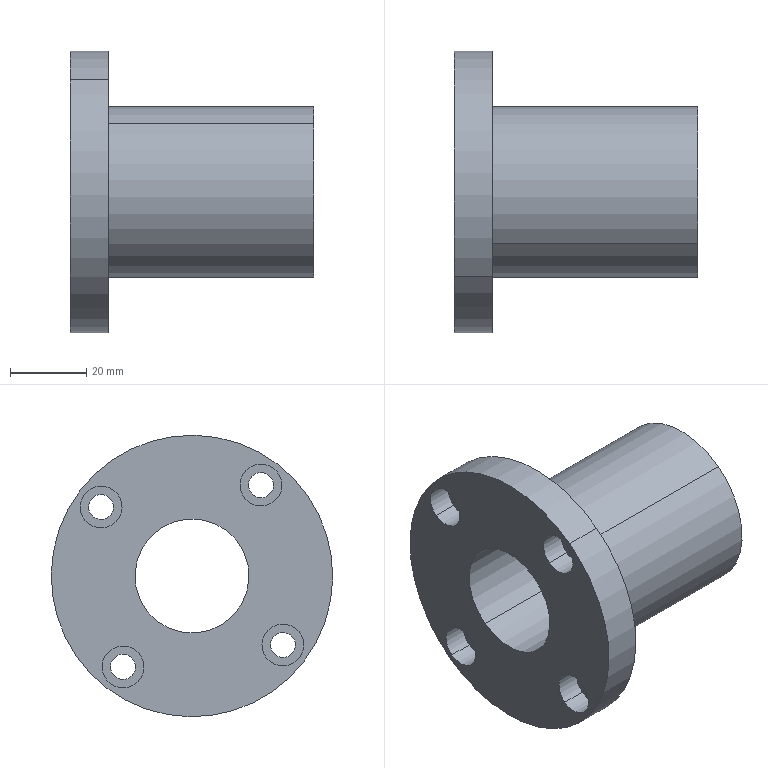Component | SolidWorks | 30LinearBearing-1 | 1 solid | 29 faces | box 64 x 74 x 74 mm | volume 80703 mm3 | cylinder 22 | plane 7 | commonest cylinder face diameters 11 x8 6.6 x8 45 x2 74 x2 30 x2
STEP:
#1=COLOUR_RGB('',0.7922,0.8196,0.9333);
#2=FILL_AREA_STYLE_COLOUR('',#1);
#3=FILL_AREA_STYLE('',(#2));
#4=SURFACE_STYLE_FILL_AREA(#3);
#5=SURFACE_SIDE_STYLE('',(#4));
#6=SURFACE_STYLE_USAGE(.BOTH.,#5);
#7=PRESENTATION_STYLE_ASSIGNMENT((#6));
#8=CARTESIAN_POINT('',(20.217,52.014,25.938));
#9=VERTEX_POINT('',#8);
#10=CARTESIAN_POINT('',(20.217,51.753,26.283));
#11=VERTEX_POINT('',#10);
#12=CARTESIAN_POINT('',(20.217,51.883,26.111));
#13=DIRECTION('',(-1.,-0.,-0.));
#14=DIRECTION('',(0.,-0.6045,0.7966));
#15=AXIS2_PLACEMENT_3D('',#12,#13,#14);
#16=CIRCLE('',#15,0.2165);
#17=EDGE_CURVE('',#9,#11,#16,.T.);
#18=ORIENTED_EDGE('',*,*,#17,.F.);
#19=CARTESIAN_POINT('',(19.961,52.014,25.938));
#20=VERTEX_POINT('',#19);
#21=CARTESIAN_POINT('',(20.217,52.014,25.938));
#22=DIRECTION('',(-1.,-0.,-0.));
#23=VECTOR('',#22,39.37);
#24=LINE('',#21,#23);
#25=EDGE_CURVE('',#9,#20,#24,.T.);
#26=ORIENTED_EDGE('',*,*,#25,.T.);
#27=CARTESIAN_POINT('',(19.961,51.753,26.283));
#28=VERTEX_POINT('',#27);
#29=CARTESIAN_POINT('',(19.961,51.883,26.111));
#30=DIRECTION('',(-1.,-0.,-0.));
#31=DIRECTION('',(0.,-0.6045,0.7966));
#32=AXIS2_PLACEMENT_3D('',#29,#30,#31);
#33=CIRCLE('',#32,0.2165);
#34=EDGE_CURVE('',#20,#28,#33,.T.);
#35=ORIENTED_EDGE('',*,*,#34,.T.);
#36=CARTESIAN_POINT('',(20.217,51.753,26.283));
#37=DIRECTION('',(-1.,-0.,-0.));
#38=VECTOR('',#37,39.37);
#39=LINE('',#36,#38);
#40=EDGE_CURVE('',#11,#28,#39,.T.);
#41=ORIENTED_EDGE('',*,*,#40,.F.);
#42=EDGE_LOOP('',(#18,#26,#35,#41));
#43=FACE_OUTER_BOUND('',#42,.T.);
#44=CARTESIAN_POINT('',(20.217,51.883,26.111));
#45=DIRECTION('',(-1.,-0.,-0.));
#46=DIRECTION('',(0.,-0.6045,0.7966));
#47=AXIS2_PLACEMENT_3D('',#44,#45,#46);
#48=CYLINDRICAL_SURFACE('',#47,0.2165);
#49=ADVANCED_FACE('',(#43),#48,.F.);
#50=CARTESIAN_POINT('',(20.217,50.36,26.165));
#51=VERTEX_POINT('',#50);
#52=CARTESIAN_POINT('',(20.217,50.098,26.51));
#53=VERTEX_POINT('',#52);
#54=CARTESIAN_POINT('',(20.217,50.229,26.338));
#55=DIRECTION('',(-1.,-0.,-0.));
#56=DIRECTION('',(0.,-0.6045,0.7966));
#57=AXIS2_PLACEMENT_3D('',#54,#55,#56);
#58=CIRCLE('',#57,0.2165);
#59=EDGE_CURVE('',#51,#53,#58,.T.);
#60=ORIENTED_EDGE('',*,*,#59,.F.);
#61=CARTESIAN_POINT('',(19.961,50.36,26.165));
#62=VERTEX_POINT('',#61);
#63=CARTESIAN_POINT('',(20.217,50.36,26.165));
#64=DIRECTION('',(-1.,-0.,-0.));
#65=VECTOR('',#64,39.37);
#66=LINE('',#63,#65);
#67=EDGE_CURVE('',#51,#62,#66,.T.);
#68=ORIENTED_EDGE('',*,*,#67,.T.);
#69=CARTESIAN_POINT('',(19.961,50.098,26.51));
#70=VERTEX_POINT('',#69);
#71=CARTESIAN_POINT('',(19.961,50.229,26.338));
#72=DIRECTION('',(-1.,-0.,-0.));
#73=DIRECTION('',(0.,-0.6045,0.7966));
#74=AXIS2_PLACEMENT_3D('',#71,#72,#73);
#75=CIRCLE('',#74,0.2165);
#76=EDGE_CURVE('',#62,#70,#75,.T.);
#77=ORIENTED_EDGE('',*,*,#76,.T.);
#78=CARTESIAN_POINT('',(20.217,50.098,26.51));
#79=DIRECTION('',(-1.,-0.,-0.));
#80=VECTOR('',#79,39.37);
#81=LINE('',#78,#80);
#82=EDGE_CURVE('',#53,#70,#81,.T.);
#83=ORIENTED_EDGE('',*,*,#82,.F.);
#84=EDGE_LOOP('',(#60,#68,#77,#83));
#85=FACE_OUTER_BOUND('',#84,.T.);
#86=CARTESIAN_POINT('',(20.217,50.229,26.338));
#87=DIRECTION('',(-1.,-0.,-0.));
#88=DIRECTION('',(0.,-0.6045,0.7966));
#89=AXIS2_PLACEMENT_3D('',#86,#87,#88);
#90=CYLINDRICAL_SURFACE('',#89,0.2165);
#91=ADVANCED_FACE('',(#85),#90,.F.);
#92=CARTESIAN_POINT('',(20.217,50.586,27.82));
#93=VERTEX_POINT('',#92);
#94=CARTESIAN_POINT('',(20.217,50.325,28.165));
#95=VERTEX_POINT('',#94);
#96=CARTESIAN_POINT('',(20.217,50.456,27.993));
#97=DIRECTION('',(-1.,-0.,-0.));
#98=DIRECTION('',(0.,-0.6045,0.7966));
#99=AXIS2_PLACEMENT_3D('',#96,#97,#98);
#100=CIRCLE('',#99,0.2165);
#101=EDGE_CURVE('',#93,#95,#100,.T.);
#102=ORIENTED_EDGE('',*,*,#101,.F.);
#103=CARTESIAN_POINT('',(19.961,50.586,27.82));
#104=VERTEX_POINT('',#103);
#105=CARTESIAN_POINT('',(20.217,50.586,27.82));
#106=DIRECTION('',(-1.,-0.,-0.));
#107=VECTOR('',#106,39.37);
#108=LINE('',#105,#107);
#109=EDGE_CURVE('',#93,#104,#108,.T.);
#110=ORIENTED_EDGE('',*,*,#109,.T.);
#111=CARTESIAN_POINT('',(19.961,50.325,28.165));
#112=VERTEX_POINT('',#111);
#113=CARTESIAN_POINT('',(19.961,50.456,27.993));
#114=DIRECTION('',(-1.,-0.,-0.));
#115=DIRECTION('',(0.,-0.6045,0.7966));
#116=AXIS2_PLACEMENT_3D('',#113,#114,#115);
#117=CIRCLE('',#116,0.2165);
#118=EDGE_CURVE('',#104,#112,#117,.T.);
#119=ORIENTED_EDGE('',*,*,#118,.T.);
#120=CARTESIAN_POINT('',(20.217,50.325,28.165));
#121=DIRECTION('',(-1.,-0.,-0.));
#122=VECTOR('',#121,39.37);
#123=LINE('',#120,#122);
#124=EDGE_CURVE('',#95,#112,#123,.T.);
#125=ORIENTED_EDGE('',*,*,#124,.F.);
#126=EDGE_LOOP('',(#102,#110,#119,#125));
#127=FACE_OUTER_BOUND('',#126,.T.);
#128=CARTESIAN_POINT('',(20.217,50.456,27.993));
#129=DIRECTION('',(-1.,-0.,-0.));
#130=DIRECTION('',(0.,-0.6045,0.7966));
#131=AXIS2_PLACEMENT_3D('',#128,#129,#130);
#132=CYLINDRICAL_SURFACE('',#131,0.2165);
#133=ADVANCED_FACE('',(#127),#132,.F.);
#134=CARTESIAN_POINT('',(20.217,52.241,27.593));
#135=VERTEX_POINT('',#134);
#136=CARTESIAN_POINT('',(20.217,51.98,27.938));
#137=VERTEX_POINT('',#136);
#138=CARTESIAN_POINT('',(20.217,52.11,27.766));
#139=DIRECTION('',(-1.,-0.,-0.));
#140=DIRECTION('',(0.,-0.6045,0.7966));
#141=AXIS2_PLACEMENT_3D('',#138,#139,#140);
#142=CIRCLE('',#141,0.2165);
#143=EDGE_CURVE('',#135,#137,#142,.T.);
#144=ORIENTED_EDGE('',*,*,#143,.F.);
#145=CARTESIAN_POINT('',(19.961,52.241,27.593));
#146=VERTEX_POINT('',#145);
#147=CARTESIAN_POINT('',(20.217,52.241,27.593));
#148=DIRECTION('',(-1.,-0.,-0.));
#149=VECTOR('',#148,39.37);
#150=LINE('',#147,#149);
#151=EDGE_CURVE('',#135,#146,#150,.T.);
#152=ORIENTED_EDGE('',*,*,#151,.T.);
#153=CARTESIAN_POINT('',(19.961,51.98,27.938));
#154=VERTEX_POINT('',#153);
#155=CARTESIAN_POINT('',(19.961,52.11,27.766));
#156=DIRECTION('',(-1.,-0.,-0.));
#157=DIRECTION('',(0.,-0.6045,0.7966));
#158=AXIS2_PLACEMENT_3D('',#155,#156,#157);
#159=CIRCLE('',#158,0.2165);
#160=EDGE_CURVE('',#146,#154,#159,.T.);
#161=ORIENTED_EDGE('',*,*,#160,.T.);
#162=CARTESIAN_POINT('',(20.217,51.98,27.938));
#163=DIRECTION('',(-1.,-0.,-0.));
#164=VECTOR('',#163,39.37);
#165=LINE('',#162,#164);
#166=EDGE_CURVE('',#137,#154,#165,.T.);
#167=ORIENTED_EDGE('',*,*,#166,.F.);
#168=EDGE_LOOP('',(#144,#152,#161,#167));
#169=FACE_OUTER_BOUND('',#168,.T.);
#170=CARTESIAN_POINT('',(20.217,52.11,27.766));
#171=DIRECTION('',(-1.,-0.,-0.));
#172=DIRECTION('',(0.,-0.6045,0.7966));
#173=AXIS2_PLACEMENT_3D('',#170,#171,#172);
#174=CYLINDRICAL_SURFACE('',#173,0.2165);
#175=ADVANCED_FACE('',(#169),#174,.F.);
#176=CARTESIAN_POINT('',(22.48,50.634,27.757));
#177=VERTEX_POINT('',#176);
#178=CARTESIAN_POINT('',(22.48,51.705,26.346));
#179=VERTEX_POINT('',#178);
#180=CARTESIAN_POINT('',(22.48,51.17,27.052));
#181=DIRECTION('',(-1.,-0.,-0.));
#182=DIRECTION('',(0.,-0.6045,0.7966));
#183=AXIS2_PLACEMENT_3D('',#180,#181,#182);
#184=CIRCLE('',#183,0.8858);
#185=EDGE_CURVE('',#177,#179,#184,.T.);
#186=ORIENTED_EDGE('',*,*,#185,.T.);
#187=CARTESIAN_POINT('',(20.354,51.705,26.346));
#188=VERTEX_POINT('',#187);
#189=CARTESIAN_POINT('',(17.576,51.705,26.346));
#190=DIRECTION('',(-1.,-0.,-0.));
#191=VECTOR('',#190,39.37);
#192=LINE('',#189,#191);
#193=EDGE_CURVE('',#179,#188,#192,.T.);
#194=ORIENTED_EDGE('',*,*,#193,.T.);
#195=CARTESIAN_POINT('',(20.354,50.634,27.757));
#196=VERTEX_POINT('',#195);
#197=CARTESIAN_POINT('',(20.354,51.17,27.052));
#198=DIRECTION('',(-1.,-0.,-0.));
#199=DIRECTION('',(0.,-0.6045,0.7966));
#200=AXIS2_PLACEMENT_3D('',#197,#198,#199);
#201=CIRCLE('',#200,0.8858);
#202=EDGE_CURVE('',#196,#188,#201,.T.);
#203=ORIENTED_EDGE('',*,*,#202,.F.);
#204=CARTESIAN_POINT('',(17.576,50.634,27.757));
#205=DIRECTION('',(-1.,-0.,-0.));
#206=VECTOR('',#205,39.37);
#207=LINE('',#204,#206);
#208=EDGE_CURVE('',#177,#196,#207,.T.);
#209=ORIENTED_EDGE('',*,*,#208,.F.);
#210=EDGE_LOOP('',(#186,#194,#203,#209));
#211=FACE_OUTER_BOUND('',#210,.T.);
#212=CARTESIAN_POINT('',(17.576,51.17,27.052));
#213=DIRECTION('',(-1.,-0.,-0.));
#214=DIRECTION('',(0.,-0.6045,0.7966));
#215=AXIS2_PLACEMENT_3D('',#212,#213,#214);
#216=CYLINDRICAL_SURFACE('',#215,0.8858);
#217=ADVANCED_FACE('',(#211),#216,.T.);
#218=CARTESIAN_POINT('',(20.354,50.289,28.212));
#219=VERTEX_POINT('',#218);
#220=CARTESIAN_POINT('',(20.354,52.05,25.891));
#221=VERTEX_POINT('',#220);
#222=CARTESIAN_POINT('',(20.354,51.17,27.052));
#223=DIRECTION('',(-1.,-0.,-0.));
#224=DIRECTION('',(0.,-0.6045,0.7966));
#225=AXIS2_PLACEMENT_3D('',#222,#223,#224);
#226=CIRCLE('',#225,1.457);
#227=EDGE_CURVE('',#219,#221,#226,.T.);
#228=ORIENTED_EDGE('',*,*,#227,.T.);
#229=CARTESIAN_POINT('',(19.961,52.05,25.891));
#230=VERTEX_POINT('',#229);
#231=CARTESIAN_POINT('',(17.576,52.05,25.891));
#232=DIRECTION('',(-1.,-0.,-0.));
#233=VECTOR('',#232,39.37);
#234=LINE('',#231,#233);
#235=EDGE_CURVE('',#221,#230,#234,.T.);
#236=ORIENTED_EDGE('',*,*,#235,.T.);
#237=CARTESIAN_POINT('',(19.961,50.289,28.212));
#238=VERTEX_POINT('',#237);
#239=CARTESIAN_POINT('',(19.961,51.17,27.052));
#240=DIRECTION('',(-1.,-0.,-0.));
#241=DIRECTION('',(0.,-0.6045,0.7966));
#242=AXIS2_PLACEMENT_3D('',#239,#240,#241);
#243=CIRCLE('',#242,1.457);
#244=EDGE_CURVE('',#238,#230,#243,.T.);
#245=ORIENTED_EDGE('',*,*,#244,.F.);
#246=CARTESIAN_POINT('',(17.576,50.289,28.212));
#247=DIRECTION('',(-1.,-0.,-0.));
#248=VECTOR('',#247,39.37);
#249=LINE('',#246,#248);
#250=EDGE_CURVE('',#219,#238,#249,.T.);
#251=ORIENTED_EDGE('',*,*,#250,.F.);
#252=EDGE_LOOP('',(#228,#236,#245,#251));
#253=FACE_OUTER_BOUND('',#252,.T.);
#254=CARTESIAN_POINT('',(17.576,51.17,27.052));
#255=DIRECTION('',(-1.,-0.,-0.));
#256=DIRECTION('',(0.,-0.6045,0.7966));
#257=AXIS2_PLACEMENT_3D('',#254,#255,#256);
#258=CYLINDRICAL_SURFACE('',#257,1.457);
#259=ADVANCED_FACE('',(#253),#258,.T.);
#260=CARTESIAN_POINT('',(22.48,51.526,26.581));
#261=VERTEX_POINT('',#260);
#262=CARTESIAN_POINT('',(22.48,50.813,27.522));
#263=VERTEX_POINT('',#262);
#264=CARTESIAN_POINT('',(22.48,51.17,27.052));
#265=DIRECTION('',(-1.,-0.,-0.));
#266=DIRECTION('',(0.,-0.6045,0.7966));
#267=AXIS2_PLACEMENT_3D('',#264,#265,#266);
#268=CIRCLE('',#267,0.5906);
#269=EDGE_CURVE('',#261,#263,#268,.T.);
#270=ORIENTED_EDGE('',*,*,#269,.F.);
#271=CARTESIAN_POINT('',(19.961,51.526,26.581));
#272=VERTEX_POINT('',#271);
#273=CARTESIAN_POINT('',(17.576,51.526,26.581));
#274=DIRECTION('',(-1.,-0.,-0.));
#275=VECTOR('',#274,39.37);
#276=LINE('',#273,#275);
#277=EDGE_CURVE('',#261,#272,#276,.T.);
#278=ORIENTED_EDGE('',*,*,#277,.T.);
#279=CARTESIAN_POINT('',(19.961,50.813,27.522));
#280=VERTEX_POINT('',#279);
#281=CARTESIAN_POINT('',(19.961,51.17,27.052));
#282=DIRECTION('',(-1.,-0.,-0.));
#283=DIRECTION('',(0.,-0.6045,0.7966));
#284=AXIS2_PLACEMENT_3D('',#281,#282,#283);
#285=CIRCLE('',#284,0.5906);
#286=EDGE_CURVE('',#272,#280,#285,.T.);
#287=ORIENTED_EDGE('',*,*,#286,.T.);
#288=CARTESIAN_POINT('',(17.576,50.813,27.522));
#289=DIRECTION('',(-1.,-0.,-0.));
#290=VECTOR('',#289,39.37);
#291=LINE('',#288,#290);
#292=EDGE_CURVE('',#263,#280,#291,.T.);
#293=ORIENTED_EDGE('',*,*,#292,.F.);
#294=EDGE_LOOP('',(#270,#278,#287,#293));
#295=FACE_OUTER_BOUND('',#294,.T.);
#296=CARTESIAN_POINT('',(17.576,51.17,27.052));
#297=DIRECTION('',(-1.,-0.,-0.));
#298=DIRECTION('',(0.,-0.6045,0.7966));
#299=AXIS2_PLACEMENT_3D('',#296,#297,#298);
#300=CYLINDRICAL_SURFACE('',#299,0.5906);
#301=ADVANCED_FACE('',(#295),#300,.F.);
#302=CARTESIAN_POINT('',(20.354,52.189,27.662));
#303=VERTEX_POINT('',#302);
#304=CARTESIAN_POINT('',(20.354,52.032,27.869));
#305=VERTEX_POINT('',#304);
#306=CARTESIAN_POINT('',(20.354,52.11,27.766));
#307=DIRECTION('',(-1.,-0.,-0.));
#308=DIRECTION('',(0.,-0.6045,0.7966));
#309=AXIS2_PLACEMENT_3D('',#306,#307,#308);
#310=CIRCLE('',#309,0.1299);
#311=EDGE_CURVE('',#303,#305,#310,.T.);
#312=ORIENTED_EDGE('',*,*,#311,.F.);
#313=CARTESIAN_POINT('',(20.217,52.189,27.662));
#314=VERTEX_POINT('',#313);
#315=CARTESIAN_POINT('',(22.48,52.189,27.662));
#316=DIRECTION('',(-1.,-0.,-0.));
#317=VECTOR('',#316,39.37);
#318=LINE('',#315,#317);
#319=EDGE_CURVE('',#303,#314,#318,.T.);
#320=ORIENTED_EDGE('',*,*,#319,.T.);
#321=CARTESIAN_POINT('',(20.217,52.032,27.869));
#322=VERTEX_POINT('',#321);
#323=CARTESIAN_POINT('',(20.217,52.11,27.766));
#324=DIRECTION('',(1.,0.,0.));
#325=DIRECTION('',(0.,-0.6045,0.7966));
#326=AXIS2_PLACEMENT_3D('',#323,#324,#325);
#327=CIRCLE('',#326,0.1299);
#328=EDGE_CURVE('',#322,#314,#327,.T.);
#329=ORIENTED_EDGE('',*,*,#328,.F.);
#330=CARTESIAN_POINT('',(22.48,52.032,27.869));
#331=DIRECTION('',(-1.,-0.,-0.));
#332=VECTOR('',#331,39.37);
#333=LINE('',#330,#332);
#334=EDGE_CURVE('',#305,#322,#333,.T.);
#335=ORIENTED_EDGE('',*,*,#334,.F.);
#336=EDGE_LOOP('',(#312,#320,#329,#335));
#337=FACE_OUTER_BOUND('',#336,.T.);
#338=CARTESIAN_POINT('',(22.48,52.11,27.766));
#339=DIRECTION('',(-1.,-0.,-0.));
#340=DIRECTION('',(0.,-0.6045,0.7966));
#341=AXIS2_PLACEMENT_3D('',#338,#339,#340);
#342=CYLINDRICAL_SURFACE('',#341,0.1299);
#343=ADVANCED_FACE('',(#337),#342,.F.);
#344=CARTESIAN_POINT('',(20.354,50.534,27.889));
#345=VERTEX_POINT('',#344);
#346=CARTESIAN_POINT('',(20.354,50.377,28.096));
#347=VERTEX_POINT('',#346);
#348=CARTESIAN_POINT('',(20.354,50.456,27.993));
#349=DIRECTION('',(-1.,-0.,-0.));
#350=DIRECTION('',(0.,-0.6045,0.7966));
#351=AXIS2_PLACEMENT_3D('',#348,#349,#350);
#352=CIRCLE('',#351,0.1299);
#353=EDGE_CURVE('',#345,#347,#352,.T.);
#354=ORIENTED_EDGE('',*,*,#353,.F.);
#355=CARTESIAN_POINT('',(20.217,50.534,27.889));
#356=VERTEX_POINT('',#355);
#357=CARTESIAN_POINT('',(22.48,50.534,27.889));
#358=DIRECTION('',(-1.,-0.,-0.));
#359=VECTOR('',#358,39.37);
#360=LINE('',#357,#359);
#361=EDGE_CURVE('',#345,#356,#360,.T.);
#362=ORIENTED_EDGE('',*,*,#361,.T.);
#363=CARTESIAN_POINT('',(20.217,50.377,28.096));
#364=VERTEX_POINT('',#363);
#365=CARTESIAN_POINT('',(20.217,50.456,27.993));
#366=DIRECTION('',(1.,0.,0.));
#367=DIRECTION('',(0.,-0.6045,0.7966));
#368=AXIS2_PLACEMENT_3D('',#365,#366,#367);
#369=CIRCLE('',#368,0.1299);
#370=EDGE_CURVE('',#364,#356,#369,.T.);
#371=ORIENTED_EDGE('',*,*,#370,.F.);
#372=CARTESIAN_POINT('',(22.48,50.377,28.096));
#373=DIRECTION('',(-1.,-0.,-0.));
#374=VECTOR('',#373,39.37);
#375=LINE('',#372,#374);
#376=EDGE_CURVE('',#347,#364,#375,.T.);
#377=ORIENTED_EDGE('',*,*,#376,.F.);
#378=EDGE_LOOP('',(#354,#362,#371,#377));
#379=FACE_OUTER_BOUND('',#378,.T.);
#380=CARTESIAN_POINT('',(22.48,50.456,27.993));
#381=DIRECTION('',(-1.,-0.,-0.));
#382=DIRECTION('',(0.,-0.6045,0.7966));
#383=AXIS2_PLACEMENT_3D('',#380,#381,#382);
#384=CYLINDRICAL_SURFACE('',#383,0.1299);
#385=ADVANCED_FACE('',(#379),#384,.F.);
#386=CARTESIAN_POINT('',(20.354,50.307,26.234));
#387=VERTEX_POINT('',#386);
#388=CARTESIAN_POINT('',(20.354,50.15,26.441));
#389=VERTEX_POINT('',#388);
#390=CARTESIAN_POINT('',(20.354,50.229,26.338));
#391=DIRECTION('',(-1.,-0.,-0.));
#392=DIRECTION('',(0.,-0.6045,0.7966));
#393=AXIS2_PLACEMENT_3D('',#390,#391,#392);
#394=CIRCLE('',#393,0.1299);
#395=EDGE_CURVE('',#387,#389,#394,.T.);
#396=ORIENTED_EDGE('',*,*,#395,.F.);
#397=CARTESIAN_POINT('',(20.217,50.307,26.234));
#398=VERTEX_POINT('',#397);
#399=CARTESIAN_POINT('',(22.48,50.307,26.234));
#400=DIRECTION('',(-1.,-0.,-0.));
#401=VECTOR('',#400,39.37);
#402=LINE('',#399,#401);
#403=EDGE_CURVE('',#387,#398,#402,.T.);
#404=ORIENTED_EDGE('',*,*,#403,.T.);
#405=CARTESIAN_POINT('',(20.217,50.15,26.441));
#406=VERTEX_POINT('',#405);
#407=CARTESIAN_POINT('',(20.217,50.229,26.338));
#408=DIRECTION('',(1.,0.,0.));
#409=DIRECTION('',(0.,-0.6045,0.7966));
#410=AXIS2_PLACEMENT_3D('',#407,#408,#409);
#411=CIRCLE('',#410,0.1299);
#412=EDGE_CURVE('',#406,#398,#411,.T.);
#413=ORIENTED_EDGE('',*,*,#412,.F.);
#414=CARTESIAN_POINT('',(22.48,50.15,26.441));
#415=DIRECTION('',(-1.,-0.,-0.));
#416=VECTOR('',#415,39.37);
#417=LINE('',#414,#416);
#418=EDGE_CURVE('',#389,#406,#417,.T.);
#419=ORIENTED_EDGE('',*,*,#418,.F.);
#420=EDGE_LOOP('',(#396,#404,#413,#419));
#421=FACE_OUTER_BOUND('',#420,.T.);
#422=CARTESIAN_POINT('',(22.48,50.229,26.338));
#423=DIRECTION('',(-1.,-0.,-0.));
#424=DIRECTION('',(0.,-0.6045,0.7966));
#425=AXIS2_PLACEMENT_3D('',#422,#423,#424);
#426=CYLINDRICAL_SURFACE('',#425,0.1299);
#427=ADVANCED_FACE('',(#421),#426,.F.);
#428=CARTESIAN_POINT('',(20.354,51.962,26.007));
#429=VERTEX_POINT('',#428);
#430=CARTESIAN_POINT('',(20.354,51.805,26.214));
#431=VERTEX_POINT('',#430);
#432=CARTESIAN_POINT('',(20.354,51.883,26.111));
#433=DIRECTION('',(-1.,-0.,-0.));
#434=DIRECTION('',(0.,-0.6045,0.7966));
#435=AXIS2_PLACEMENT_3D('',#432,#433,#434);
#436=CIRCLE('',#435,0.1299);
#437=EDGE_CURVE('',#429,#431,#436,.T.);
#438=ORIENTED_EDGE('',*,*,#437,.F.);
#439=CARTESIAN_POINT('',(20.217,51.962,26.007));
#440=VERTEX_POINT('',#439);
#441=CARTESIAN_POINT('',(22.48,51.962,26.007));
#442=DIRECTION('',(-1.,-0.,-0.));
#443=VECTOR('',#442,39.37);
#444=LINE('',#441,#443);
#445=EDGE_CURVE('',#429,#440,#444,.T.);
#446=ORIENTED_EDGE('',*,*,#445,.T.);
#447=CARTESIAN_POINT('',(20.217,51.805,26.214));
#448=VERTEX_POINT('',#447);
#449=CARTESIAN_POINT('',(20.217,51.883,26.111));
#450=DIRECTION('',(1.,0.,0.));
#451=DIRECTION('',(0.,-0.6045,0.7966));
#452=AXIS2_PLACEMENT_3D('',#449,#450,#451);
#453=CIRCLE('',#452,0.1299);
#454=EDGE_CURVE('',#448,#440,#453,.T.);
#455=ORIENTED_EDGE('',*,*,#454,.F.);
#456=CARTESIAN_POINT('',(22.48,51.805,26.214));
#457=DIRECTION('',(-1.,-0.,-0.));
#458=VECTOR('',#457,39.37);
#459=LINE('',#456,#458);
#460=EDGE_CURVE('',#431,#448,#459,.T.);
#461=ORIENTED_EDGE('',*,*,#460,.F.);
#462=EDGE_LOOP('',(#438,#446,#455,#461));
#463=FACE_OUTER_BOUND('',#462,.T.);
#464=CARTESIAN_POINT('',(22.48,51.883,26.111));
#465=DIRECTION('',(-1.,-0.,-0.));
#466=DIRECTION('',(0.,-0.6045,0.7966));
#467=AXIS2_PLACEMENT_3D('',#464,#465,#466);
#468=CYLINDRICAL_SURFACE('',#467,0.1299);
#469=ADVANCED_FACE('',(#463),#468,.F.);
#470=ORIENTED_EDGE('',*,*,#445,.F.);
#471=CARTESIAN_POINT('',(20.354,51.883,26.111));
#472=DIRECTION('',(-1.,-0.,-0.));
#473=DIRECTION('',(0.,-0.6045,0.7966));
#474=AXIS2_PLACEMENT_3D('',#471,#472,#473);
#475=CIRCLE('',#474,0.1299);
#476=EDGE_CURVE('',#431,#429,#475,.T.);
#477=ORIENTED_EDGE('',*,*,#476,.F.);
#478=ORIENTED_EDGE('',*,*,#460,.T.);
#479=CARTESIAN_POINT('',(20.217,51.883,26.111));
#480=DIRECTION('',(1.,0.,0.));
#481=DIRECTION('',(0.,-0.6045,0.7966));
#482=AXIS2_PLACEMENT_3D('',#479,#480,#481);
#483=CIRCLE('',#482,0.1299);
#484=EDGE_CURVE('',#440,#448,#483,.T.);
#485=ORIENTED_EDGE('',*,*,#484,.F.);
#486=EDGE_LOOP('',(#470,#477,#478,#485));
#487=FACE_OUTER_BOUND('',#486,.T.);
#488=CARTESIAN_POINT('',(22.48,51.883,26.111));
#489=DIRECTION('',(-1.,-0.,-0.));
#490=DIRECTION('',(0.,-0.6045,0.7966));
#491=AXIS2_PLACEMENT_3D('',#488,#489,#490);
#492=CYLINDRICAL_SURFACE('',#491,0.1299);
#493=ADVANCED_FACE('',(#487),#492,.F.);
#494=ORIENTED_EDGE('',*,*,#403,.F.);
#495=CARTESIAN_POINT('',(20.354,50.229,26.338));
#496=DIRECTION('',(-1.,-0.,-0.));
#497=DIRECTION('',(0.,-0.6045,0.7966));
#498=AXIS2_PLACEMENT_3D('',#495,#496,#497);
#499=CIRCLE('',#498,0.1299);
#500=EDGE_CURVE('',#389,#387,#499,.T.);
#501=ORIENTED_EDGE('',*,*,#500,.F.);
#502=ORIENTED_EDGE('',*,*,#418,.T.);
#503=CARTESIAN_POINT('',(20.217,50.229,26.338));
#504=DIRECTION('',(1.,0.,0.));
#505=DIRECTION('',(0.,-0.6045,0.7966));
#506=AXIS2_PLACEMENT_3D('',#503,#504,#505);
#507=CIRCLE('',#506,0.1299);
#508=EDGE_CURVE('',#398,#406,#507,.T.);
#509=ORIENTED_EDGE('',*,*,#508,.F.);
#510=EDGE_LOOP('',(#494,#501,#502,#509));
#511=FACE_OUTER_BOUND('',#510,.T.);
#512=CARTESIAN_POINT('',(22.48,50.229,26.338));
#513=DIRECTION('',(-1.,-0.,-0.));
#514=DIRECTION('',(0.,-0.6045,0.7966));
#515=AXIS2_PLACEMENT_3D('',#512,#513,#514);
#516=CYLINDRICAL_SURFACE('',#515,0.1299);
#517=ADVANCED_FACE('',(#511),#516,.F.);
#518=ORIENTED_EDGE('',*,*,#361,.F.);
#519=CARTESIAN_POINT('',(20.354,50.456,27.993));
#520=DIRECTION('',(-1.,-0.,-0.));
#521=DIRECTION('',(0.,-0.6045,0.7966));
#522=AXIS2_PLACEMENT_3D('',#519,#520,#521);
#523=CIRCLE('',#522,0.1299);
#524=EDGE_CURVE('',#347,#345,#523,.T.);
#525=ORIENTED_EDGE('',*,*,#524,.F.);
#526=ORIENTED_EDGE('',*,*,#376,.T.);
#527=CARTESIAN_POINT('',(20.217,50.456,27.993));
#528=DIRECTION('',(1.,0.,0.));
#529=DIRECTION('',(0.,-0.6045,0.7966));
#530=AXIS2_PLACEMENT_3D('',#527,#528,#529);
#531=CIRCLE('',#530,0.1299);
#532=EDGE_CURVE('',#356,#364,#531,.T.);
#533=ORIENTED_EDGE('',*,*,#532,.F.);
#534=EDGE_LOOP('',(#518,#525,#526,#533));
#535=FACE_OUTER_BOUND('',#534,.T.);
#536=CARTESIAN_POINT('',(22.48,50.456,27.993));
#537=DIRECTION('',(-1.,-0.,-0.));
#538=DIRECTION('',(0.,-0.6045,0.7966));
#539=AXIS2_PLACEMENT_3D('',#536,#537,#538);
#540=CYLINDRICAL_SURFACE('',#539,0.1299);
#541=ADVANCED_FACE('',(#535),#540,.F.);
#542=ORIENTED_EDGE('',*,*,#319,.F.);
#543=CARTESIAN_POINT('',(20.354,52.11,27.766));
#544=DIRECTION('',(-1.,-0.,-0.));
#545=DIRECTION('',(0.,-0.6045,0.7966));
#546=AXIS2_PLACEMENT_3D('',#543,#544,#545);
#547=CIRCLE('',#546,0.1299);
#548=EDGE_CURVE('',#305,#303,#547,.T.);
#549=ORIENTED_EDGE('',*,*,#548,.F.);
#550=ORIENTED_EDGE('',*,*,#334,.T.);
#551=CARTESIAN_POINT('',(20.217,52.11,27.766));
#552=DIRECTION('',(1.,0.,0.));
#553=DIRECTION('',(0.,-0.6045,0.7966));
#554=AXIS2_PLACEMENT_3D('',#551,#552,#553);
#555=CIRCLE('',#554,0.1299);
#556=EDGE_CURVE('',#314,#322,#555,.T.);
#557=ORIENTED_EDGE('',*,*,#556,.F.);
#558=EDGE_LOOP('',(#542,#549,#550,#557));
#559=FACE_OUTER_BOUND('',#558,.T.);
#560=CARTESIAN_POINT('',(22.48,52.11,27.766));
#561=DIRECTION('',(-1.,-0.,-0.));
#562=DIRECTION('',(0.,-0.6045,0.7966));
#563=AXIS2_PLACEMENT_3D('',#560,#561,#562);
#564=CYLINDRICAL_SURFACE('',#563,0.1299);
#565=ADVANCED_FACE('',(#559),#564,.F.);
#566=ORIENTED_EDGE('',*,*,#277,.F.);
#567=CARTESIAN_POINT('',(22.48,51.17,27.052));
#568=DIRECTION('',(-1.,-0.,-0.));
#569=DIRECTION('',(0.,-0.6045,0.7966));
#570=AXIS2_PLACEMENT_3D('',#567,#568,#569);
#571=CIRCLE('',#570,0.5906);
#572=EDGE_CURVE('',#263,#261,#571,.T.);
#573=ORIENTED_EDGE('',*,*,#572,.F.);
#574=ORIENTED_EDGE('',*,*,#292,.T.);
#575=CARTESIAN_POINT('',(19.961,51.17,27.052));
#576=DIRECTION('',(-1.,-0.,-0.));
#577=DIRECTION('',(0.,-0.6045,0.7966));
#578=AXIS2_PLACEMENT_3D('',#575,#576,#577);
#579=CIRCLE('',#578,0.5906);
#580=EDGE_CURVE('',#280,#272,#579,.T.);
#581=ORIENTED_EDGE('',*,*,#580,.T.);
#582=EDGE_LOOP('',(#566,#573,#574,#581));
#583=FACE_OUTER_BOUND('',#582,.T.);
#584=CARTESIAN_POINT('',(17.576,51.17,27.052));
#585=DIRECTION('',(-1.,-0.,-0.));
#586=DIRECTION('',(0.,-0.6045,0.7966));
#587=AXIS2_PLACEMENT_3D('',#584,#585,#586);
#588=CYLINDRICAL_SURFACE('',#587,0.5906);
#589=ADVANCED_FACE('',(#583),#588,.F.);
#590=CARTESIAN_POINT('',(19.961,51.883,26.111));
#591=DIRECTION('',(-1.,-0.,-0.));
#592=DIRECTION('',(0.,-0.6045,0.7966));
#593=AXIS2_PLACEMENT_3D('',#590,#591,#592);
#594=CIRCLE('',#593,0.2165);
#595=EDGE_CURVE('',#28,#20,#594,.T.);
#596=ORIENTED_EDGE('',*,*,#595,.F.);
#597=ORIENTED_EDGE('',*,*,#34,.F.);
#598=EDGE_LOOP('',(#596,#597));
#599=FACE_BOUND('',#598,.T.);
#600=CARTESIAN_POINT('',(19.961,50.229,26.338));
#601=DIRECTION('',(-1.,-0.,-0.));
#602=DIRECTION('',(0.,-0.6045,0.7966));
#603=AXIS2_PLACEMENT_3D('',#600,#601,#602);
#604=CIRCLE('',#603,0.2165);
#605=EDGE_CURVE('',#70,#62,#604,.T.);
#606=ORIENTED_EDGE('',*,*,#605,.F.);
#607=ORIENTED_EDGE('',*,*,#76,.F.);
#608=EDGE_LOOP('',(#606,#607));
#609=FACE_BOUND('',#608,.T.);
#610=CARTESIAN_POINT('',(19.961,50.456,27.993));
#611=DIRECTION('',(-1.,-0.,-0.));
#612=DIRECTION('',(0.,-0.6045,0.7966));
#613=AXIS2_PLACEMENT_3D('',#610,#611,#612);
#614=CIRCLE('',#613,0.2165);
#615=EDGE_CURVE('',#112,#104,#614,.T.);
#616=ORIENTED_EDGE('',*,*,#615,.F.);
#617=ORIENTED_EDGE('',*,*,#118,.F.);
#618=EDGE_LOOP('',(#616,#617));
#619=FACE_BOUND('',#618,.T.);
#620=CARTESIAN_POINT('',(19.961,52.11,27.766));
#621=DIRECTION('',(-1.,-0.,-0.));
#622=DIRECTION('',(0.,-0.6045,0.7966));
#623=AXIS2_PLACEMENT_3D('',#620,#621,#622);
#624=CIRCLE('',#623,0.2165);
#625=EDGE_CURVE('',#154,#146,#624,.T.);
#626=ORIENTED_EDGE('',*,*,#625,.F.);
#627=ORIENTED_EDGE('',*,*,#160,.F.);
#628=EDGE_LOOP('',(#626,#627));
#629=FACE_BOUND('',#628,.T.);
#630=ORIENTED_EDGE('',*,*,#580,.F.);
#631=ORIENTED_EDGE('',*,*,#286,.F.);
#632=EDGE_LOOP('',(#630,#631));
#633=FACE_BOUND('',#632,.T.);
#634=ORIENTED_EDGE('',*,*,#244,.T.);
#635=CARTESIAN_POINT('',(19.961,51.17,27.052));
#636=DIRECTION('',(-1.,-0.,-0.));
#637=DIRECTION('',(0.,-0.6045,0.7966));
#638=AXIS2_PLACEMENT_3D('',#635,#636,#637);
#639=CIRCLE('',#638,1.457);
#640=EDGE_CURVE('',#230,#238,#639,.T.);
#641=ORIENTED_EDGE('',*,*,#640,.T.);
#642=EDGE_LOOP('',(#634,#641));
#643=FACE_OUTER_BOUND('',#642,.T.);
#644=CARTESIAN_POINT('',(19.961,51.64,27.409));
#645=DIRECTION('',(1.,0.,0.));
#646=DIRECTION('',(-0.,0.6045,-0.7966));
#647=AXIS2_PLACEMENT_3D('',#644,#645,#646);
#648=PLANE('',#647);
#649=ADVANCED_FACE('',(#599,#609,#619,#629,#633,#643),#648,.F.);
#650=ORIENTED_EDGE('',*,*,#235,.F.);
#651=CARTESIAN_POINT('',(20.354,51.17,27.052));
#652=DIRECTION('',(-1.,-0.,-0.));
#653=DIRECTION('',(0.,-0.6045,0.7966));
#654=AXIS2_PLACEMENT_3D('',#651,#652,#653);
#655=CIRCLE('',#654,1.457);
#656=EDGE_CURVE('',#221,#219,#655,.T.);
#657=ORIENTED_EDGE('',*,*,#656,.T.);
#658=ORIENTED_EDGE('',*,*,#250,.T.);
#659=ORIENTED_EDGE('',*,*,#640,.F.);
#660=EDGE_LOOP('',(#650,#657,#658,#659));
#661=FACE_OUTER_BOUND('',#660,.T.);
#662=CARTESIAN_POINT('',(17.576,51.17,27.052));
#663=DIRECTION('',(-1.,-0.,-0.));
#664=DIRECTION('',(0.,-0.6045,0.7966));
#665=AXIS2_PLACEMENT_3D('',#662,#663,#664);
#666=CYLINDRICAL_SURFACE('',#665,1.457);
#667=ADVANCED_FACE('',(#661),#666,.T.);
#668=ORIENTED_EDGE('',*,*,#476,.T.);
#669=ORIENTED_EDGE('',*,*,#437,.T.);
#670=EDGE_LOOP('',(#668,#669));
#671=FACE_BOUND('',#670,.T.);
#672=ORIENTED_EDGE('',*,*,#500,.T.);
#673=ORIENTED_EDGE('',*,*,#395,.T.);
#674=EDGE_LOOP('',(#672,#673));
#675=FACE_BOUND('',#674,.T.);
#676=ORIENTED_EDGE('',*,*,#524,.T.);
#677=ORIENTED_EDGE('',*,*,#353,.T.);
#678=EDGE_LOOP('',(#676,#677));
#679=FACE_BOUND('',#678,.T.);
#680=ORIENTED_EDGE('',*,*,#548,.T.);
#681=ORIENTED_EDGE('',*,*,#311,.T.);
#682=EDGE_LOOP('',(#680,#681));
#683=FACE_BOUND('',#682,.T.);
#684=ORIENTED_EDGE('',*,*,#227,.F.);
#685=ORIENTED_EDGE('',*,*,#656,.F.);
#686=EDGE_LOOP('',(#684,#685));
#687=FACE_OUTER_BOUND('',#686,.T.);
#688=ORIENTED_EDGE('',*,*,#202,.T.);
#689=CARTESIAN_POINT('',(20.354,51.17,27.052));
#690=DIRECTION('',(-1.,-0.,-0.));
#691=DIRECTION('',(0.,-0.6045,0.7966));
#692=AXIS2_PLACEMENT_3D('',#689,#690,#691);
#693=CIRCLE('',#692,0.8858);
#694=EDGE_CURVE('',#188,#196,#693,.T.);
#695=ORIENTED_EDGE('',*,*,#694,.T.);
#696=EDGE_LOOP('',(#688,#695));
#697=FACE_BOUND('',#696,.T.);
#698=CARTESIAN_POINT('',(20.354,52.33,27.932));
#699=DIRECTION('',(-1.,-0.,-0.));
#700=DIRECTION('',(0.,-0.6045,0.7966));
#701=AXIS2_PLACEMENT_3D('',#698,#699,#700);
#702=PLANE('',#701);
#703=ADVANCED_FACE('',(#671,#675,#679,#683,#687,#697),#702,.F.);
#704=ORIENTED_EDGE('',*,*,#193,.F.);
#705=CARTESIAN_POINT('',(22.48,51.17,27.052));
#706=DIRECTION('',(-1.,-0.,-0.));
#707=DIRECTION('',(0.,-0.6045,0.7966));
#708=AXIS2_PLACEMENT_3D('',#705,#706,#707);
#709=CIRCLE('',#708,0.8858);
#710=EDGE_CURVE('',#179,#177,#709,.T.);
#711=ORIENTED_EDGE('',*,*,#710,.T.);
#712=ORIENTED_EDGE('',*,*,#208,.T.);
#713=ORIENTED_EDGE('',*,*,#694,.F.);
#714=EDGE_LOOP('',(#704,#711,#712,#713));
#715=FACE_OUTER_BOUND('',#714,.T.);
#716=CARTESIAN_POINT('',(17.576,51.17,27.052));
#717=DIRECTION('',(-1.,-0.,-0.));
#718=DIRECTION('',(0.,-0.6045,0.7966));
#719=AXIS2_PLACEMENT_3D('',#716,#717,#718);
#720=CYLINDRICAL_SURFACE('',#719,0.8858);
#721=ADVANCED_FACE('',(#715),#720,.T.);
#722=ORIENTED_EDGE('',*,*,#185,.F.);
#723=ORIENTED_EDGE('',*,*,#710,.F.);
#724=EDGE_LOOP('',(#722,#723));
#725=FACE_OUTER_BOUND('',#724,.T.);
#726=ORIENTED_EDGE('',*,*,#572,.T.);
#727=ORIENTED_EDGE('',*,*,#269,.T.);
#728=EDGE_LOOP('',(#726,#727));
#729=FACE_BOUND('',#728,.T.);
#730=CARTESIAN_POINT('',(22.48,51.875,27.587));
#731=DIRECTION('',(-1.,-0.,-0.));
#732=DIRECTION('',(0.,-0.6045,0.7966));
#733=AXIS2_PLACEMENT_3D('',#730,#731,#732);
#734=PLANE('',#733);
#735=ADVANCED_FACE('',(#725,#729),#734,.F.);
#736=CARTESIAN_POINT('',(20.217,52.11,27.766));
#737=DIRECTION('',(-1.,-0.,-0.));
#738=DIRECTION('',(0.,-0.6045,0.7966));
#739=AXIS2_PLACEMENT_3D('',#736,#737,#738);
#740=CIRCLE('',#739,0.2165);
#741=EDGE_CURVE('',#137,#135,#740,.T.);
#742=ORIENTED_EDGE('',*,*,#741,.T.);
#743=ORIENTED_EDGE('',*,*,#143,.T.);
#744=EDGE_LOOP('',(#742,#743));
#745=FACE_OUTER_BOUND('',#744,.T.);
#746=ORIENTED_EDGE('',*,*,#328,.T.);
#747=ORIENTED_EDGE('',*,*,#556,.T.);
#748=EDGE_LOOP('',(#746,#747));
#749=FACE_BOUND('',#748,.T.);
#750=CARTESIAN_POINT('',(20.217,52.11,27.766));
#751=DIRECTION('',(-1.,-0.,-0.));
#752=DIRECTION('',(0.,-0.6045,0.7966));
#753=AXIS2_PLACEMENT_3D('',#750,#751,#752);
#754=PLANE('',#753);
#755=ADVANCED_FACE('',(#745,#749),#754,.T.);
#756=ORIENTED_EDGE('',*,*,#151,.F.);
#757=ORIENTED_EDGE('',*,*,#741,.F.);
#758=ORIENTED_EDGE('',*,*,#166,.T.);
#759=ORIENTED_EDGE('',*,*,#625,.T.);
#760=EDGE_LOOP('',(#756,#757,#758,#759));
#761=FACE_OUTER_BOUND('',#760,.T.);
#762=CARTESIAN_POINT('',(20.217,52.11,27.766));
#763=DIRECTION('',(-1.,-0.,-0.));
#764=DIRECTION('',(0.,-0.6045,0.7966));
#765=AXIS2_PLACEMENT_3D('',#762,#763,#764);
#766=CYLINDRICAL_SURFACE('',#765,0.2165);
#767=ADVANCED_FACE('',(#761),#766,.F.);
#768=CARTESIAN_POINT('',(20.217,50.456,27.993));
#769=DIRECTION('',(-1.,-0.,-0.));
#770=DIRECTION('',(0.,-0.6045,0.7966));
#771=AXIS2_PLACEMENT_3D('',#768,#769,#770);
#772=CIRCLE('',#771,0.2165);
#773=EDGE_CURVE('',#95,#93,#772,.T.);
#774=ORIENTED_EDGE('',*,*,#773,.T.);
#775=ORIENTED_EDGE('',*,*,#101,.T.);
#776=EDGE_LOOP('',(#774,#775));
#777=FACE_OUTER_BOUND('',#776,.T.);
#778=ORIENTED_EDGE('',*,*,#370,.T.);
#779=ORIENTED_EDGE('',*,*,#532,.T.);
#780=EDGE_LOOP('',(#778,#779));
#781=FACE_BOUND('',#780,.T.);
#782=CARTESIAN_POINT('',(20.217,50.456,27.993));
#783=DIRECTION('',(-1.,-0.,-0.));
#784=DIRECTION('',(0.,-0.6045,0.7966));
#785=AXIS2_PLACEMENT_3D('',#782,#783,#784);
#786=PLANE('',#785);
#787=ADVANCED_FACE('',(#777,#781),#786,.T.);
#788=ORIENTED_EDGE('',*,*,#109,.F.);
#789=ORIENTED_EDGE('',*,*,#773,.F.);
#790=ORIENTED_EDGE('',*,*,#124,.T.);
#791=ORIENTED_EDGE('',*,*,#615,.T.);
#792=EDGE_LOOP('',(#788,#789,#790,#791));
#793=FACE_OUTER_BOUND('',#792,.T.);
#794=CARTESIAN_POINT('',(20.217,50.456,27.993));
#795=DIRECTION('',(-1.,-0.,-0.));
#796=DIRECTION('',(0.,-0.6045,0.7966));
#797=AXIS2_PLACEMENT_3D('',#794,#795,#796);
#798=CYLINDRICAL_SURFACE('',#797,0.2165);
#799=ADVANCED_FACE('',(#793),#798,.F.);
#800=CARTESIAN_POINT('',(20.217,50.229,26.338));
#801=DIRECTION('',(-1.,-0.,-0.));
#802=DIRECTION('',(0.,-0.6045,0.7966));
#803=AXIS2_PLACEMENT_3D('',#800,#801,#802);
#804=CIRCLE('',#803,0.2165);
#805=EDGE_CURVE('',#53,#51,#804,.T.);
#806=ORIENTED_EDGE('',*,*,#805,.T.);
#807=ORIENTED_EDGE('',*,*,#59,.T.);
#808=EDGE_LOOP('',(#806,#807));
#809=FACE_OUTER_BOUND('',#808,.T.);
#810=ORIENTED_EDGE('',*,*,#412,.T.);
#811=ORIENTED_EDGE('',*,*,#508,.T.);
#812=EDGE_LOOP('',(#810,#811));
#813=FACE_BOUND('',#812,.T.);
#814=CARTESIAN_POINT('',(20.217,50.229,26.338));
#815=DIRECTION('',(-1.,-0.,-0.));
#816=DIRECTION('',(0.,-0.6045,0.7966));
#817=AXIS2_PLACEMENT_3D('',#814,#815,#816);
#818=PLANE('',#817);
#819=ADVANCED_FACE('',(#809,#813),#818,.T.);
#820=ORIENTED_EDGE('',*,*,#67,.F.);
#821=ORIENTED_EDGE('',*,*,#805,.F.);
#822=ORIENTED_EDGE('',*,*,#82,.T.);
#823=ORIENTED_EDGE('',*,*,#605,.T.);
#824=EDGE_LOOP('',(#820,#821,#822,#823));
#825=FACE_OUTER_BOUND('',#824,.T.);
#826=CARTESIAN_POINT('',(20.217,50.229,26.338));
#827=DIRECTION('',(-1.,-0.,-0.));
#828=DIRECTION('',(0.,-0.6045,0.7966));
#829=AXIS2_PLACEMENT_3D('',#826,#827,#828);
#830=CYLINDRICAL_SURFACE('',#829,0.2165);
#831=ADVANCED_FACE('',(#825),#830,.F.);
#832=CARTESIAN_POINT('',(20.217,51.883,26.111));
#833=DIRECTION('',(-1.,-0.,-0.));
#834=DIRECTION('',(0.,-0.6045,0.7966));
#835=AXIS2_PLACEMENT_3D('',#832,#833,#834);
#836=CIRCLE('',#835,0.2165);
#837=EDGE_CURVE('',#11,#9,#836,.T.);
#838=ORIENTED_EDGE('',*,*,#837,.T.);
#839=ORIENTED_EDGE('',*,*,#17,.T.);
#840=EDGE_LOOP('',(#838,#839));
#841=FACE_OUTER_BOUND('',#840,.T.);
#842=ORIENTED_EDGE('',*,*,#454,.T.);
#843=ORIENTED_EDGE('',*,*,#484,.T.);
#844=EDGE_LOOP('',(#842,#843));
#845=FACE_BOUND('',#844,.T.);
#846=CARTESIAN_POINT('',(20.217,51.883,26.111));
#847=DIRECTION('',(-1.,-0.,-0.));
#848=DIRECTION('',(0.,-0.6045,0.7966));
#849=AXIS2_PLACEMENT_3D('',#846,#847,#848);
#850=PLANE('',#849);
#851=ADVANCED_FACE('',(#841,#845),#850,.T.);
#852=ORIENTED_EDGE('',*,*,#25,.F.);
#853=ORIENTED_EDGE('',*,*,#837,.F.);
#854=ORIENTED_EDGE('',*,*,#40,.T.);
#855=ORIENTED_EDGE('',*,*,#595,.T.);
#856=EDGE_LOOP('',(#852,#853,#854,#855));
#857=FACE_OUTER_BOUND('',#856,.T.);
#858=CARTESIAN_POINT('',(20.217,51.883,26.111));
#859=DIRECTION('',(-1.,-0.,-0.));
#860=DIRECTION('',(0.,-0.6045,0.7966));
#861=AXIS2_PLACEMENT_3D('',#858,#859,#860);
#862=CYLINDRICAL_SURFACE('',#861,0.2165);
#863=ADVANCED_FACE('',(#857),#862,.F.);
#864=CLOSED_SHELL('',(#49,#91,#133,#175,#217,#259,#301,#343,#385,#427,#469,#493,#517,#541,#565,#589,#649,#667,#703,#721,#735,#755,#767,#787,#799,#819,#831,#851,#863));
#865=MANIFOLD_SOLID_BREP('',#864);
#866=STYLED_ITEM('',(#7),#865);
#867=(LENGTH_UNIT()NAMED_UNIT(*)SI_UNIT($,.METRE.));
#868=LENGTH_MEASURE_WITH_UNIT(LENGTH_MEASURE(0.0254),#867);
#869=DIMENSIONAL_EXPONENTS(1.,0.,0.,0.,0.,0.,0.);
#870=(CONVERSION_BASED_UNIT('',#868)LENGTH_UNIT()NAMED_UNIT(#869));
#871=UNCERTAINTY_MEASURE_WITH_UNIT(LENGTH_MEASURE(0.00001),#870,'','');
#872=(NAMED_UNIT(*)PLANE_ANGLE_UNIT()SI_UNIT($,.RADIAN.));
#873=(NAMED_UNIT(*)SI_UNIT($,.STERADIAN.)SOLID_ANGLE_UNIT());
#874=(GEOMETRIC_REPRESENTATION_CONTEXT(3)GLOBAL_UNCERTAINTY_ASSIGNED_CONTEXT((#871))GLOBAL_UNIT_ASSIGNED_CONTEXT((#870,#872,#873))REPRESENTATION_CONTEXT('',''));
#875=MECHANICAL_DESIGN_GEOMETRIC_PRESENTATION_REPRESENTATION('',(#866),#874);
#876=CARTESIAN_POINT('',(0.,0.,0.));
#877=DIRECTION('',(0.,0.,1.));
#878=DIRECTION('',(1.,0.,0.));
#879=AXIS2_PLACEMENT_3D('',#876,#877,#878);
#880=(LENGTH_UNIT()NAMED_UNIT(*)SI_UNIT($,.METRE.));
#881=LENGTH_MEASURE_WITH_UNIT(LENGTH_MEASURE(0.0254),#880);
#882=DIMENSIONAL_EXPONENTS(1.,0.,0.,0.,0.,0.,0.);
#883=(CONVERSION_BASED_UNIT('',#881)LENGTH_UNIT()NAMED_UNIT(#882));
#884=UNCERTAINTY_MEASURE_WITH_UNIT(LENGTH_MEASURE(0.00001),#883,'','');
#885=(NAMED_UNIT(*)PLANE_ANGLE_UNIT()SI_UNIT($,.RADIAN.));
#886=(NAMED_UNIT(*)SI_UNIT($,.STERADIAN.)SOLID_ANGLE_UNIT());
#887=(GEOMETRIC_REPRESENTATION_CONTEXT(3)GLOBAL_UNCERTAINTY_ASSIGNED_CONTEXT((#884))GLOBAL_UNIT_ASSIGNED_CONTEXT((#883,#885,#886))REPRESENTATION_CONTEXT('',''));
#888=ADVANCED_BREP_SHAPE_REPRESENTATION('',(#865,#879),#887);
#889=PRESENTATION_LAYER_ASSIGNMENT('','',(#866));